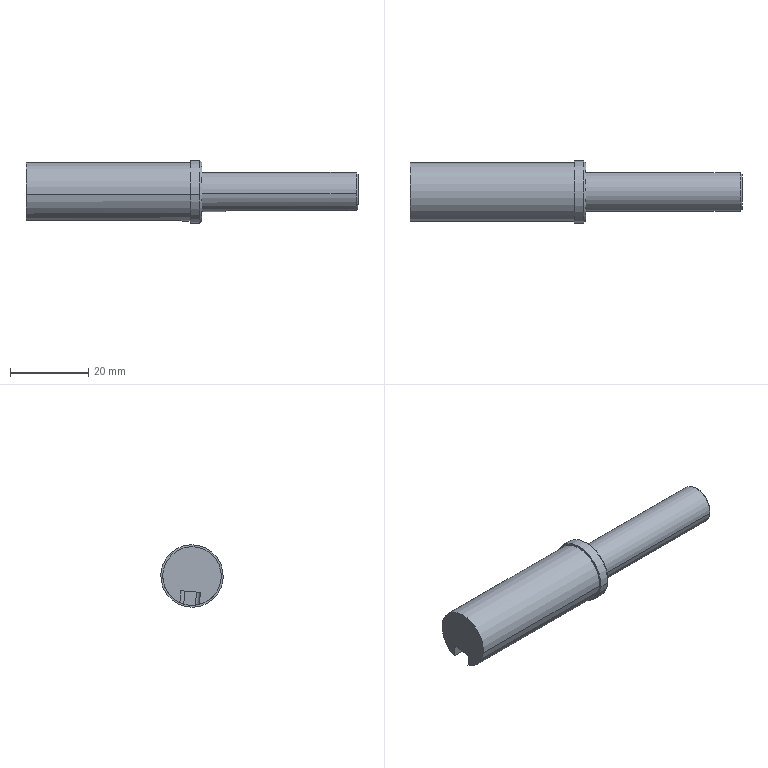Component | SolidWorks | 2018SOLIDWORKS1000000020-1 | 1 solid | 31 faces | box 85 x 16 x 16 mm | volume 10078 mm3 | cylinder 12 | plane 12 | cone 7 | commonest cylinder face diameters 2 x4 15 x2 3.3 x2 10 x2 16 x2 | material 45 Steel
build123d program:
from build123d import *

# Parameters (mm, degrees)
SKETCH1_R             = 8
BOSS_EXTRUDE1_DEPTH   = 45
SKETCH3_R             = 5
BOSS_EXTRUDE3_DEPTH   = 40
CHAMFER1_SIZE         = 0.5
M4_TAPPED_HOLE1_D     = 3.3
M4_TAPPED_HOLE1_DEPTH = 10
M4_TAPPED_HOLE1_TIP   = 0.9914
CHAMFER2_SIZE         = 0.5
SKETCH9_R             = 10
SKETCH9_R_2           = 7.5
CUT_EXTRUDE1_DEPTH    = 42
SKETCH10_W            = 5
SKETCH10_H            = 5
CUT_EXTRUDE2_DEPTH    = 40
FILLET1_R             = 1
SKETCH11_W            = 4
SKETCH11_H            = 4
CUT_EXTRUDE3_DEPTH    = 34
FILLET2_R             = 1


with BuildPart() as part:
    # Sketch1 → Boss-Extrude1 (new body)
    with BuildSketch(Plane.XY):
        with Locations(Location((0, 0, 0), (0, 0, 180))):
            Circle(SKETCH1_R)
    extrude(amount=BOSS_EXTRUDE1_DEPTH)

    # Sketch3 → Boss-Extrude3 (add)
    with BuildSketch(Plane.XY.offset(45)):
        Circle(SKETCH3_R)
    extrude(amount=BOSS_EXTRUDE3_DEPTH)

    # Chamfer1
    chamfer1_edges = [part.edges().sort_by_distance(p)[0] for p in [
        (8, 0, 0),
        (8, 0, 45),
    ]]
    chamfer(chamfer1_edges, length=CHAMFER1_SIZE)

    # M4 Tapped Hole1
    with Locations(Plane(origin=(0, 0, 85), x_dir=(-1, 0, 0), z_dir=(0, 0, 1))):
        with Locations((0, 0)):
            Hole(M4_TAPPED_HOLE1_D / 2, depth=M4_TAPPED_HOLE1_DEPTH)
            with Locations((0, 0, -(M4_TAPPED_HOLE1_DEPTH + M4_TAPPED_HOLE1_TIP / 2))):  # 118° drill point
                Cone(0, M4_TAPPED_HOLE1_D / 2, M4_TAPPED_HOLE1_TIP, mode=Mode.SUBTRACT)

    # Chamfer2
    chamfer2_edges = [part.edges().sort_by_distance(p)[0] for p in [
        (-5, 0, 85),
    ]]
    chamfer(chamfer2_edges, length=CHAMFER2_SIZE)

    # Sketch9 → Cut-Extrude1 (cut)
    with BuildSketch(Plane(origin=(0, 0, 0), x_dir=(-1, 0, 0), z_dir=(0, 0, -1))):
        Circle(SKETCH9_R)
        Circle(SKETCH9_R_2, mode=Mode.SUBTRACT)
    extrude(amount=-CUT_EXTRUDE1_DEPTH, mode=Mode.SUBTRACT)

    # Sketch10 → Cut-Extrude2 (cut)
    with BuildSketch(Plane(origin=(0, 0, 0), x_dir=(-1, 0, 0), z_dir=(0, 0, -1))):
        with Locations((0, 6.5)):
            Rectangle(SKETCH10_W, SKETCH10_H)
    extrude(amount=-CUT_EXTRUDE2_DEPTH, mode=Mode.SUBTRACT)

    # Fillet1
    fillet1_edges = [part.edges().sort_by_distance(p)[0] for p in [
        (2.5, 5.536, 40),
        (-2.5, 5.536, 40),
    ]]
    fillet(fillet1_edges, radius=FILLET1_R)

    # Sketch11 → Cut-Extrude3 (cut)
    with BuildSketch(Plane.XY.offset(85)):
        with Locations((0, 4.5)):
            Rectangle(SKETCH11_W, SKETCH11_H)
    extrude(amount=-CUT_EXTRUDE3_DEPTH, mode=Mode.SUBTRACT)

    # Fillet2
    fillet2_edges = [part.edges().sort_by_distance(p)[0] for p in [
        (-2, 3.541, 51),
        (2, 3.541, 51),
    ]]
    fillet(fillet2_edges, radius=FILLET2_R)


solid = part.part

# Placed as in the assembly
solid = solid.moved(Location((-72.284, -95.825, 207.018), (-85.06, 90, 0)))
STEP:
#1=COLOUR_RGB('',0.7922,0.8196,0.9333);
#2=FILL_AREA_STYLE_COLOUR('',#1);
#3=FILL_AREA_STYLE('',(#2));
#4=SURFACE_STYLE_FILL_AREA(#3);
#5=SURFACE_SIDE_STYLE('',(#4));
#6=SURFACE_STYLE_USAGE(.BOTH.,#5);
#7=PRESENTATION_STYLE_ASSIGNMENT((#6));
#8=CARTESIAN_POINT('',(-1.192,-3.478,8.176));
#9=VERTEX_POINT('',#8);
#10=CARTESIAN_POINT('',(-1.192,-4.067,8.125));
#11=VERTEX_POINT('',#10);
#12=CARTESIAN_POINT('',(-1.192,-3.773,8.15));
#13=DIRECTION('',(-1.,-0.,0.));
#14=DIRECTION('',(0.,-0.9963,-0.08611));
#15=AXIS2_PLACEMENT_3D('',#12,#13,#14);
#16=CIRCLE('',#15,0.2953);
#17=EDGE_CURVE('',#9,#11,#16,.T.);
#18=ORIENTED_EDGE('',*,*,#17,.T.);
#19=CARTESIAN_POINT('',(-2.846,-4.067,8.125));
#20=VERTEX_POINT('',#19);
#21=CARTESIAN_POINT('',(0.03939,-4.067,8.125));
#22=DIRECTION('',(-1.,-0.,0.));
#23=VECTOR('',#22,39.37);
#24=LINE('',#21,#23);
#25=EDGE_CURVE('',#11,#20,#24,.T.);
#26=ORIENTED_EDGE('',*,*,#25,.T.);
#27=CARTESIAN_POINT('',(-2.846,-3.847,7.864));
#28=VERTEX_POINT('',#27);
#29=CARTESIAN_POINT('',(-2.846,-3.773,8.15));
#30=DIRECTION('',(-1.,-0.,0.));
#31=DIRECTION('',(0.,0.9963,0.08611));
#32=AXIS2_PLACEMENT_3D('',#29,#30,#31);
#33=CIRCLE('',#32,0.2953);
#34=EDGE_CURVE('',#28,#20,#33,.T.);
#35=ORIENTED_EDGE('',*,*,#34,.F.);
#36=CARTESIAN_POINT('',(-1.31,-3.847,7.864));
#37=VERTEX_POINT('',#36);
#38=CARTESIAN_POINT('',(0.03939,-3.847,7.864));
#39=DIRECTION('',(-1.,-0.,0.));
#40=VECTOR('',#39,39.37);
#41=LINE('',#38,#40);
#42=EDGE_CURVE('',#37,#28,#41,.T.);
#43=ORIENTED_EDGE('',*,*,#42,.F.);
#44=CARTESIAN_POINT('',(-1.271,-3.807,7.857));
#45=VERTEX_POINT('',#44);
#46=CARTESIAN_POINT('',(-1.31,-3.847,7.864));
#47=CARTESIAN_POINT('',(-1.305,-3.847,7.864));
#48=CARTESIAN_POINT('',(-1.3,-3.846,7.864));
#49=CARTESIAN_POINT('',(-1.29,-3.841,7.863));
#50=CARTESIAN_POINT('',(-1.286,-3.838,7.862));
#51=CARTESIAN_POINT('',(-1.279,-3.831,7.861));
#52=CARTESIAN_POINT('',(-1.276,-3.827,7.86));
#53=CARTESIAN_POINT('',(-1.272,-3.817,7.858));
#54=CARTESIAN_POINT('',(-1.271,-3.812,7.858));
#55=CARTESIAN_POINT('',(-1.271,-3.807,7.857));
#56=B_SPLINE_CURVE_WITH_KNOTS('',3,(#46,#47,#48,#49,#50,#51,#52,#53,#54,#55),.UNSPECIFIED.,.F.,.F.,(4,2,2,2,4),(0.,0.0003975,0.000795,0.001193,0.00159),.UNSPECIFIED.);
#57=EDGE_CURVE('',#37,#45,#56,.T.);
#58=ORIENTED_EDGE('',*,*,#57,.T.);
#59=CARTESIAN_POINT('',(-1.271,-3.689,7.867));
#60=VERTEX_POINT('',#59);
#61=CARTESIAN_POINT('',(-1.271,-3.773,8.15));
#62=DIRECTION('',(1.,0.,-0.));
#63=DIRECTION('',(0.,0.9963,0.08611));
#64=AXIS2_PLACEMENT_3D('',#61,#62,#63);
#65=CIRCLE('',#64,0.2953);
#66=EDGE_CURVE('',#45,#60,#65,.T.);
#67=ORIENTED_EDGE('',*,*,#66,.T.);
#68=CARTESIAN_POINT('',(-1.31,-3.651,7.881));
#69=VERTEX_POINT('',#68);
#70=CARTESIAN_POINT('',(-1.271,-3.689,7.867));
#71=CARTESIAN_POINT('',(-1.271,-3.684,7.869));
#72=CARTESIAN_POINT('',(-1.272,-3.679,7.87));
#73=CARTESIAN_POINT('',(-1.276,-3.67,7.874));
#74=CARTESIAN_POINT('',(-1.279,-3.665,7.875));
#75=CARTESIAN_POINT('',(-1.286,-3.658,7.878));
#76=CARTESIAN_POINT('',(-1.29,-3.656,7.879));
#77=CARTESIAN_POINT('',(-1.3,-3.652,7.881));
#78=CARTESIAN_POINT('',(-1.305,-3.651,7.881));
#79=CARTESIAN_POINT('',(-1.31,-3.651,7.881));
#80=B_SPLINE_CURVE_WITH_KNOTS('',3,(#70,#71,#72,#73,#74,#75,#76,#77,#78,#79),.UNSPECIFIED.,.F.,.F.,(4,2,2,2,4),(0.,0.0003975,0.000795,0.001193,0.00159),.UNSPECIFIED.);
#81=EDGE_CURVE('',#60,#69,#80,.T.);
#82=ORIENTED_EDGE('',*,*,#81,.T.);
#83=CARTESIAN_POINT('',(-2.846,-3.651,7.881));
#84=VERTEX_POINT('',#83);
#85=CARTESIAN_POINT('',(0.03939,-3.651,7.881));
#86=DIRECTION('',(1.,0.,-0.));
#87=VECTOR('',#86,39.37);
#88=LINE('',#85,#87);
#89=EDGE_CURVE('',#84,#69,#88,.T.);
#90=ORIENTED_EDGE('',*,*,#89,.F.);
#91=CARTESIAN_POINT('',(-2.846,-3.478,8.176));
#92=VERTEX_POINT('',#91);
#93=CARTESIAN_POINT('',(-2.846,-3.773,8.15));
#94=DIRECTION('',(-1.,-0.,0.));
#95=DIRECTION('',(0.,0.9963,0.08611));
#96=AXIS2_PLACEMENT_3D('',#93,#94,#95);
#97=CIRCLE('',#96,0.2953);
#98=EDGE_CURVE('',#92,#84,#97,.T.);
#99=ORIENTED_EDGE('',*,*,#98,.F.);
#100=CARTESIAN_POINT('',(0.03939,-3.478,8.176));
#101=DIRECTION('',(-1.,-0.,0.));
#102=VECTOR('',#101,39.37);
#103=LINE('',#100,#102);
#104=EDGE_CURVE('',#9,#92,#103,.T.);
#105=ORIENTED_EDGE('',*,*,#104,.F.);
#106=EDGE_LOOP('',(#18,#26,#35,#43,#58,#67,#82,#90,#99,#105));
#107=FACE_OUTER_BOUND('',#106,.T.);
#108=CARTESIAN_POINT('',(0.03939,-3.773,8.15));
#109=DIRECTION('',(-1.,-0.,0.));
#110=DIRECTION('',(-0.,0.9963,0.08611));
#111=AXIS2_PLACEMENT_3D('',#108,#109,#110);
#112=CYLINDRICAL_SURFACE('',#111,0.2953);
#113=ADVANCED_FACE('',(#107),#112,.T.);
#114=CARTESIAN_POINT('',(0.5006,-3.949,8.135));
#115=VERTEX_POINT('',#114);
#116=CARTESIAN_POINT('',(0.5006,-3.837,7.985));
#117=VERTEX_POINT('',#116);
#118=CARTESIAN_POINT('',(0.5006,-3.773,8.15));
#119=DIRECTION('',(1.,0.,-0.));
#120=DIRECTION('',(0.,-0.9963,-0.08611));
#121=AXIS2_PLACEMENT_3D('',#118,#119,#120);
#122=CIRCLE('',#121,0.1772);
#123=EDGE_CURVE('',#115,#117,#122,.T.);
#124=ORIENTED_EDGE('',*,*,#123,.F.);
#125=CARTESIAN_POINT('',(0.481,-3.969,8.133));
#126=VERTEX_POINT('',#125);
#127=CARTESIAN_POINT('',(0.5006,-3.949,8.135));
#128=DIRECTION('',(-0.7071,-0.7045,-0.06089));
#129=VECTOR('',#128,39.37);
#130=LINE('',#127,#129);
#131=EDGE_CURVE('',#115,#126,#130,.T.);
#132=ORIENTED_EDGE('',*,*,#131,.T.);
#133=CARTESIAN_POINT('',(0.481,-3.836,7.964));
#134=VERTEX_POINT('',#133);
#135=CARTESIAN_POINT('',(0.481,-3.773,8.15));
#136=DIRECTION('',(-1.,-0.,0.));
#137=DIRECTION('',(0.,-0.9963,-0.08611));
#138=AXIS2_PLACEMENT_3D('',#135,#136,#137);
#139=CIRCLE('',#138,0.1969);
#140=EDGE_CURVE('',#134,#126,#139,.T.);
#141=ORIENTED_EDGE('',*,*,#140,.F.);
#142=CARTESIAN_POINT('',(0.5006,-3.837,7.985));
#143=CARTESIAN_POINT('',(0.4941,-3.837,7.978));
#144=CARTESIAN_POINT('',(0.4876,-3.836,7.971));
#145=CARTESIAN_POINT('',(0.481,-3.836,7.964));
#146=B_SPLINE_CURVE_WITH_KNOTS('',3,(#142,#143,#144,#145),.UNSPECIFIED.,.F.,.F.,(4,4),(0.002374,0.003118),.UNSPECIFIED.);
#147=EDGE_CURVE('',#117,#134,#146,.T.);
#148=ORIENTED_EDGE('',*,*,#147,.F.);
#149=EDGE_LOOP('',(#124,#132,#141,#148));
#150=FACE_OUTER_BOUND('',#149,.T.);
#151=CARTESIAN_POINT('',(0.5006,-3.773,8.15));
#152=DIRECTION('',(-1.,-0.,0.));
#153=DIRECTION('',(-0.,0.9963,0.08611));
#154=AXIS2_PLACEMENT_3D('',#151,#152,#153);
#155=CONICAL_SURFACE('',#154,0.1772,0.7854);
#156=ADVANCED_FACE('',(#150),#155,.T.);
#157=ORIENTED_EDGE('',*,*,#131,.F.);
#158=CARTESIAN_POINT('',(0.5006,-3.596,8.166));
#159=VERTEX_POINT('',#158);
#160=CARTESIAN_POINT('',(0.5006,-3.773,8.15));
#161=DIRECTION('',(1.,0.,-0.));
#162=DIRECTION('',(0.,-0.9963,-0.08611));
#163=AXIS2_PLACEMENT_3D('',#160,#161,#162);
#164=CIRCLE('',#163,0.1772);
#165=EDGE_CURVE('',#159,#115,#164,.T.);
#166=ORIENTED_EDGE('',*,*,#165,.F.);
#167=CARTESIAN_POINT('',(0.481,-3.577,8.167));
#168=VERTEX_POINT('',#167);
#169=CARTESIAN_POINT('',(0.5006,-3.596,8.166));
#170=DIRECTION('',(-0.7071,0.7045,0.06089));
#171=VECTOR('',#170,39.37);
#172=LINE('',#169,#171);
#173=EDGE_CURVE('',#159,#168,#172,.T.);
#174=ORIENTED_EDGE('',*,*,#173,.T.);
#175=CARTESIAN_POINT('',(0.481,-3.773,8.15));
#176=DIRECTION('',(-1.,-0.,0.));
#177=DIRECTION('',(0.,-0.9963,-0.08611));
#178=AXIS2_PLACEMENT_3D('',#175,#176,#177);
#179=CIRCLE('',#178,0.1969);
#180=EDGE_CURVE('',#126,#168,#179,.T.);
#181=ORIENTED_EDGE('',*,*,#180,.F.);
#182=EDGE_LOOP('',(#157,#166,#174,#181));
#183=FACE_OUTER_BOUND('',#182,.T.);
#184=CARTESIAN_POINT('',(0.5006,-3.773,8.15));
#185=DIRECTION('',(-1.,-0.,0.));
#186=DIRECTION('',(-0.,0.9963,0.08611));
#187=AXIS2_PLACEMENT_3D('',#184,#185,#186);
#188=CONICAL_SURFACE('',#187,0.1772,0.7854);
#189=ADVANCED_FACE('',(#183),#188,.T.);
#190=CARTESIAN_POINT('',(0.1069,-3.708,8.156));
#191=VERTEX_POINT('',#190);
#192=CARTESIAN_POINT('',(0.1069,-3.837,8.145));
#193=VERTEX_POINT('',#192);
#194=CARTESIAN_POINT('',(0.1069,-3.773,8.15));
#195=DIRECTION('',(1.,0.,-0.));
#196=DIRECTION('',(0.,-0.9963,-0.08611));
#197=AXIS2_PLACEMENT_3D('',#194,#195,#196);
#198=CIRCLE('',#197,0.06496);
#199=EDGE_CURVE('',#191,#193,#198,.T.);
#200=ORIENTED_EDGE('',*,*,#199,.F.);
#201=CARTESIAN_POINT('',(0.5006,-3.708,8.156));
#202=VERTEX_POINT('',#201);
#203=CARTESIAN_POINT('',(0.5006,-3.708,8.156));
#204=DIRECTION('',(1.,0.,-0.));
#205=VECTOR('',#204,39.37);
#206=LINE('',#203,#205);
#207=EDGE_CURVE('',#191,#202,#206,.T.);
#208=ORIENTED_EDGE('',*,*,#207,.T.);
#209=CARTESIAN_POINT('',(0.5006,-3.837,8.145));
#210=VERTEX_POINT('',#209);
#211=CARTESIAN_POINT('',(0.5006,-3.773,8.15));
#212=DIRECTION('',(1.,0.,-0.));
#213=DIRECTION('',(0.,-0.9963,-0.08611));
#214=AXIS2_PLACEMENT_3D('',#211,#212,#213);
#215=CIRCLE('',#214,0.06496);
#216=EDGE_CURVE('',#202,#210,#215,.T.);
#217=ORIENTED_EDGE('',*,*,#216,.T.);
#218=CARTESIAN_POINT('',(0.5006,-3.837,8.145));
#219=DIRECTION('',(1.,0.,-0.));
#220=VECTOR('',#219,39.37);
#221=LINE('',#218,#220);
#222=EDGE_CURVE('',#193,#210,#221,.T.);
#223=ORIENTED_EDGE('',*,*,#222,.F.);
#224=EDGE_LOOP('',(#200,#208,#217,#223));
#225=FACE_OUTER_BOUND('',#224,.T.);
#226=CARTESIAN_POINT('',(0.5006,-3.773,8.15));
#227=DIRECTION('',(1.,0.,-0.));
#228=DIRECTION('',(0.,-0.9963,-0.08611));
#229=AXIS2_PLACEMENT_3D('',#226,#227,#228);
#230=CYLINDRICAL_SURFACE('',#229,0.06496);
#231=ADVANCED_FACE('',(#225),#230,.F.);
#232=CARTESIAN_POINT('',(0.06791,-3.773,8.15));
#233=VERTEX_POINT('',#232);
#234=CARTESIAN_POINT('',(0.1069,-3.837,8.145));
#235=DIRECTION('',(0.515,-0.854,-0.07381));
#236=VECTOR('',#235,39.37);
#237=LINE('',#234,#236);
#238=EDGE_CURVE('',#233,#193,#237,.T.);
#239=ORIENTED_EDGE('',*,*,#238,.F.);
#240=CARTESIAN_POINT('',(0.1069,-3.708,8.156));
#241=DIRECTION('',(0.515,0.854,0.07381));
#242=VECTOR('',#241,39.37);
#243=LINE('',#240,#242);
#244=EDGE_CURVE('',#233,#191,#243,.T.);
#245=ORIENTED_EDGE('',*,*,#244,.T.);
#246=ORIENTED_EDGE('',*,*,#199,.T.);
#247=EDGE_LOOP('',(#239,#245,#246));
#248=FACE_OUTER_BOUND('',#247,.T.);
#249=CARTESIAN_POINT('',(0.1069,-3.773,8.15));
#250=DIRECTION('',(1.,0.,-0.));
#251=DIRECTION('',(0.,-0.9963,-0.08611));
#252=AXIS2_PLACEMENT_3D('',#249,#250,#251);
#253=CONICAL_SURFACE('',#252,0.06496,1.03);
#254=ADVANCED_FACE('',(#248),#253,.F.);
#255=CARTESIAN_POINT('',(-1.074,-4.067,8.125));
#256=VERTEX_POINT('',#255);
#257=CARTESIAN_POINT('',(-1.074,-3.478,8.176));
#258=VERTEX_POINT('',#257);
#259=CARTESIAN_POINT('',(-1.074,-3.773,8.15));
#260=DIRECTION('',(1.,0.,-0.));
#261=DIRECTION('',(0.,-0.9963,-0.08611));
#262=AXIS2_PLACEMENT_3D('',#259,#260,#261);
#263=CIRCLE('',#262,0.2953);
#264=EDGE_CURVE('',#256,#258,#263,.T.);
#265=ORIENTED_EDGE('',*,*,#264,.F.);
#266=CARTESIAN_POINT('',(-1.094,-4.086,8.123));
#267=VERTEX_POINT('',#266);
#268=CARTESIAN_POINT('',(-1.074,-4.067,8.125));
#269=DIRECTION('',(-0.7071,-0.7045,-0.06089));
#270=VECTOR('',#269,39.37);
#271=LINE('',#268,#270);
#272=EDGE_CURVE('',#256,#267,#271,.T.);
#273=ORIENTED_EDGE('',*,*,#272,.T.);
#274=CARTESIAN_POINT('',(-1.094,-3.459,8.177));
#275=VERTEX_POINT('',#274);
#276=CARTESIAN_POINT('',(-1.094,-3.773,8.15));
#277=DIRECTION('',(-1.,-0.,0.));
#278=DIRECTION('',(0.,-0.9963,-0.08611));
#279=AXIS2_PLACEMENT_3D('',#276,#277,#278);
#280=CIRCLE('',#279,0.315);
#281=EDGE_CURVE('',#275,#267,#280,.T.);
#282=ORIENTED_EDGE('',*,*,#281,.F.);
#283=CARTESIAN_POINT('',(-1.074,-3.478,8.176));
#284=DIRECTION('',(-0.7071,0.7045,0.06089));
#285=VECTOR('',#284,39.37);
#286=LINE('',#283,#285);
#287=EDGE_CURVE('',#258,#275,#286,.T.);
#288=ORIENTED_EDGE('',*,*,#287,.F.);
#289=EDGE_LOOP('',(#265,#273,#282,#288));
#290=FACE_OUTER_BOUND('',#289,.T.);
#291=CARTESIAN_POINT('',(-1.074,-3.773,8.15));
#292=DIRECTION('',(-1.,-0.,0.));
#293=DIRECTION('',(-0.,0.9963,0.08611));
#294=AXIS2_PLACEMENT_3D('',#291,#292,#293);
#295=CONICAL_SURFACE('',#294,0.2953,0.7854);
#296=ADVANCED_FACE('',(#290),#295,.T.);
#297=ORIENTED_EDGE('',*,*,#140,.T.);
#298=CARTESIAN_POINT('',(-1.074,-3.969,8.133));
#299=VERTEX_POINT('',#298);
#300=CARTESIAN_POINT('',(0.5006,-3.969,8.133));
#301=DIRECTION('',(-1.,-0.,0.));
#302=VECTOR('',#301,39.37);
#303=LINE('',#300,#302);
#304=EDGE_CURVE('',#126,#299,#303,.T.);
#305=ORIENTED_EDGE('',*,*,#304,.T.);
#306=CARTESIAN_POINT('',(-1.074,-3.577,8.167));
#307=VERTEX_POINT('',#306);
#308=CARTESIAN_POINT('',(-1.074,-3.773,8.15));
#309=DIRECTION('',(1.,0.,-0.));
#310=DIRECTION('',(0.,-0.9963,-0.08611));
#311=AXIS2_PLACEMENT_3D('',#308,#309,#310);
#312=CIRCLE('',#311,0.1969);
#313=EDGE_CURVE('',#299,#307,#312,.T.);
#314=ORIENTED_EDGE('',*,*,#313,.T.);
#315=CARTESIAN_POINT('',(0.5006,-3.577,8.167));
#316=DIRECTION('',(-1.,-0.,0.));
#317=VECTOR('',#316,39.37);
#318=LINE('',#315,#317);
#319=EDGE_CURVE('',#168,#307,#318,.T.);
#320=ORIENTED_EDGE('',*,*,#319,.F.);
#321=CARTESIAN_POINT('',(0.481,-3.679,7.977));
#322=VERTEX_POINT('',#321);
#323=CARTESIAN_POINT('',(0.481,-3.773,8.15));
#324=DIRECTION('',(-1.,-0.,0.));
#325=DIRECTION('',(0.,-0.9963,-0.08611));
#326=AXIS2_PLACEMENT_3D('',#323,#324,#325);
#327=CIRCLE('',#326,0.1969);
#328=EDGE_CURVE('',#168,#322,#327,.T.);
#329=ORIENTED_EDGE('',*,*,#328,.T.);
#330=CARTESIAN_POINT('',(-0.7986,-3.679,7.977));
#331=VERTEX_POINT('',#330);
#332=CARTESIAN_POINT('',(0.5006,-3.679,7.977));
#333=DIRECTION('',(-1.,-0.,0.));
#334=VECTOR('',#333,39.37);
#335=LINE('',#332,#334);
#336=EDGE_CURVE('',#322,#331,#335,.T.);
#337=ORIENTED_EDGE('',*,*,#336,.T.);
#338=CARTESIAN_POINT('',(-0.8379,-3.717,7.962));
#339=VERTEX_POINT('',#338);
#340=CARTESIAN_POINT('',(-0.7986,-3.679,7.977));
#341=CARTESIAN_POINT('',(-0.8039,-3.679,7.977));
#342=CARTESIAN_POINT('',(-0.8091,-3.68,7.977));
#343=CARTESIAN_POINT('',(-0.8187,-3.684,7.975));
#344=CARTESIAN_POINT('',(-0.823,-3.686,7.973));
#345=CARTESIAN_POINT('',(-0.8302,-3.693,7.97));
#346=CARTESIAN_POINT('',(-0.833,-3.698,7.968));
#347=CARTESIAN_POINT('',(-0.8369,-3.707,7.965));
#348=CARTESIAN_POINT('',(-0.8379,-3.712,7.963));
#349=CARTESIAN_POINT('',(-0.8379,-3.717,7.962));
#350=B_SPLINE_CURVE_WITH_KNOTS('',3,(#340,#341,#342,#343,#344,#345,#346,#347,#348,#349),.UNSPECIFIED.,.F.,.F.,(4,2,2,2,4),(0.,0.0003995,0.0007989,0.001198,0.001598),.UNSPECIFIED.);
#351=EDGE_CURVE('',#331,#339,#350,.T.);
#352=ORIENTED_EDGE('',*,*,#351,.T.);
#353=CARTESIAN_POINT('',(-0.8379,-3.795,7.955));
#354=VERTEX_POINT('',#353);
#355=CARTESIAN_POINT('',(-0.8379,-3.773,8.15));
#356=DIRECTION('',(1.,0.,-0.));
#357=DIRECTION('',(0.,-0.9963,-0.08611));
#358=AXIS2_PLACEMENT_3D('',#355,#356,#357);
#359=CIRCLE('',#358,0.1969);
#360=EDGE_CURVE('',#354,#339,#359,.T.);
#361=ORIENTED_EDGE('',*,*,#360,.F.);
#362=CARTESIAN_POINT('',(-0.7986,-3.836,7.964));
#363=VERTEX_POINT('',#362);
#364=CARTESIAN_POINT('',(-0.8379,-3.795,7.955));
#365=CARTESIAN_POINT('',(-0.8379,-3.801,7.955));
#366=CARTESIAN_POINT('',(-0.8369,-3.806,7.956));
#367=CARTESIAN_POINT('',(-0.833,-3.815,7.958));
#368=CARTESIAN_POINT('',(-0.8302,-3.82,7.959));
#369=CARTESIAN_POINT('',(-0.823,-3.827,7.961));
#370=CARTESIAN_POINT('',(-0.8187,-3.83,7.962));
#371=CARTESIAN_POINT('',(-0.8092,-3.834,7.963));
#372=CARTESIAN_POINT('',(-0.8039,-3.836,7.964));
#373=CARTESIAN_POINT('',(-0.7986,-3.836,7.964));
#374=B_SPLINE_CURVE_WITH_KNOTS('',3,(#364,#365,#366,#367,#368,#369,#370,#371,#372,#373),.UNSPECIFIED.,.F.,.F.,(4,2,2,2,4),(0.,0.0003995,0.0007989,0.001198,0.001598),.UNSPECIFIED.);
#375=EDGE_CURVE('',#354,#363,#374,.T.);
#376=ORIENTED_EDGE('',*,*,#375,.T.);
#377=CARTESIAN_POINT('',(0.5006,-3.836,7.964));
#378=DIRECTION('',(1.,0.,-0.));
#379=VECTOR('',#378,39.37);
#380=LINE('',#377,#379);
#381=EDGE_CURVE('',#363,#134,#380,.T.);
#382=ORIENTED_EDGE('',*,*,#381,.T.);
#383=EDGE_LOOP('',(#297,#305,#314,#320,#329,#337,#352,#361,#376,#382));
#384=FACE_OUTER_BOUND('',#383,.T.);
#385=CARTESIAN_POINT('',(0.5006,-3.773,8.15));
#386=DIRECTION('',(-1.,-0.,0.));
#387=DIRECTION('',(-0.,0.9963,0.08611));
#388=AXIS2_PLACEMENT_3D('',#385,#386,#387);
#389=CYLINDRICAL_SURFACE('',#388,0.1969);
#390=ADVANCED_FACE('',(#384),#389,.T.);
#391=ORIENTED_EDGE('',*,*,#281,.T.);
#392=CARTESIAN_POINT('',(-1.192,-4.086,8.123));
#393=VERTEX_POINT('',#392);
#394=CARTESIAN_POINT('',(-1.074,-4.086,8.123));
#395=DIRECTION('',(-1.,-0.,0.));
#396=VECTOR('',#395,39.37);
#397=LINE('',#394,#396);
#398=EDGE_CURVE('',#267,#393,#397,.T.);
#399=ORIENTED_EDGE('',*,*,#398,.T.);
#400=CARTESIAN_POINT('',(-1.192,-3.459,8.177));
#401=VERTEX_POINT('',#400);
#402=CARTESIAN_POINT('',(-1.192,-3.773,8.15));
#403=DIRECTION('',(1.,0.,-0.));
#404=DIRECTION('',(0.,-0.9963,-0.08611));
#405=AXIS2_PLACEMENT_3D('',#402,#403,#404);
#406=CIRCLE('',#405,0.315);
#407=EDGE_CURVE('',#393,#401,#406,.T.);
#408=ORIENTED_EDGE('',*,*,#407,.T.);
#409=CARTESIAN_POINT('',(-1.074,-3.459,8.177));
#410=DIRECTION('',(-1.,-0.,0.));
#411=VECTOR('',#410,39.37);
#412=LINE('',#409,#411);
#413=EDGE_CURVE('',#275,#401,#412,.T.);
#414=ORIENTED_EDGE('',*,*,#413,.F.);
#415=EDGE_LOOP('',(#391,#399,#408,#414));
#416=FACE_OUTER_BOUND('',#415,.T.);
#417=CARTESIAN_POINT('',(-1.074,-3.773,8.15));
#418=DIRECTION('',(-1.,-0.,0.));
#419=DIRECTION('',(-0.,0.9963,0.08611));
#420=AXIS2_PLACEMENT_3D('',#417,#418,#419);
#421=CYLINDRICAL_SURFACE('',#420,0.315);
#422=ADVANCED_FACE('',(#416),#421,.T.);
#423=CARTESIAN_POINT('',(-1.074,-3.773,8.15));
#424=DIRECTION('',(1.,0.,-0.));
#425=DIRECTION('',(0.,-0.9963,-0.08611));
#426=AXIS2_PLACEMENT_3D('',#423,#424,#425);
#427=CIRCLE('',#426,0.2953);
#428=EDGE_CURVE('',#258,#256,#427,.T.);
#429=ORIENTED_EDGE('',*,*,#428,.T.);
#430=ORIENTED_EDGE('',*,*,#264,.T.);
#431=EDGE_LOOP('',(#429,#430));
#432=FACE_OUTER_BOUND('',#431,.T.);
#433=CARTESIAN_POINT('',(-1.074,-3.773,8.15));
#434=DIRECTION('',(1.,0.,-0.));
#435=DIRECTION('',(0.,-0.9963,-0.08611));
#436=AXIS2_PLACEMENT_3D('',#433,#434,#435);
#437=CIRCLE('',#436,0.1969);
#438=EDGE_CURVE('',#307,#299,#437,.T.);
#439=ORIENTED_EDGE('',*,*,#438,.F.);
#440=ORIENTED_EDGE('',*,*,#313,.F.);
#441=EDGE_LOOP('',(#439,#440));
#442=FACE_BOUND('',#441,.T.);
#443=CARTESIAN_POINT('',(-1.074,-3.773,8.15));
#444=DIRECTION('',(1.,0.,-0.));
#445=DIRECTION('',(0.,-0.9963,-0.08611));
#446=AXIS2_PLACEMENT_3D('',#443,#444,#445);
#447=PLANE('',#446);
#448=ADVANCED_FACE('',(#432,#442),#447,.T.);
#449=ORIENTED_EDGE('',*,*,#398,.F.);
#450=CARTESIAN_POINT('',(-1.094,-3.773,8.15));
#451=DIRECTION('',(-1.,-0.,0.));
#452=DIRECTION('',(0.,-0.9963,-0.08611));
#453=AXIS2_PLACEMENT_3D('',#450,#451,#452);
#454=CIRCLE('',#453,0.315);
#455=EDGE_CURVE('',#267,#275,#454,.T.);
#456=ORIENTED_EDGE('',*,*,#455,.T.);
#457=ORIENTED_EDGE('',*,*,#413,.T.);
#458=CARTESIAN_POINT('',(-1.192,-3.773,8.15));
#459=DIRECTION('',(1.,0.,-0.));
#460=DIRECTION('',(0.,-0.9963,-0.08611));
#461=AXIS2_PLACEMENT_3D('',#458,#459,#460);
#462=CIRCLE('',#461,0.315);
#463=EDGE_CURVE('',#401,#393,#462,.T.);
#464=ORIENTED_EDGE('',*,*,#463,.T.);
#465=EDGE_LOOP('',(#449,#456,#457,#464));
#466=FACE_OUTER_BOUND('',#465,.T.);
#467=CARTESIAN_POINT('',(-1.074,-3.773,8.15));
#468=DIRECTION('',(-1.,-0.,0.));
#469=DIRECTION('',(-0.,0.9963,0.08611));
#470=AXIS2_PLACEMENT_3D('',#467,#468,#469);
#471=CYLINDRICAL_SURFACE('',#470,0.315);
#472=ADVANCED_FACE('',(#466),#471,.T.);
#473=ORIENTED_EDGE('',*,*,#304,.F.);
#474=ORIENTED_EDGE('',*,*,#180,.T.);
#475=ORIENTED_EDGE('',*,*,#319,.T.);
#476=ORIENTED_EDGE('',*,*,#438,.T.);
#477=EDGE_LOOP('',(#473,#474,#475,#476));
#478=FACE_OUTER_BOUND('',#477,.T.);
#479=CARTESIAN_POINT('',(0.5006,-3.773,8.15));
#480=DIRECTION('',(-1.,-0.,0.));
#481=DIRECTION('',(-0.,0.9963,0.08611));
#482=AXIS2_PLACEMENT_3D('',#479,#480,#481);
#483=CYLINDRICAL_SURFACE('',#482,0.1969);
#484=ADVANCED_FACE('',(#478),#483,.T.);
#485=CARTESIAN_POINT('',(0.5006,-3.681,7.999));
#486=VERTEX_POINT('',#485);
#487=CARTESIAN_POINT('',(0.5006,-3.686,8.059));
#488=VERTEX_POINT('',#487);
#489=CARTESIAN_POINT('',(0.5006,-3.672,7.902));
#490=DIRECTION('',(0.,-0.08611,0.9963));
#491=VECTOR('',#490,39.37);
#492=LINE('',#489,#491);
#493=EDGE_CURVE('',#486,#488,#492,.T.);
#494=ORIENTED_EDGE('',*,*,#493,.F.);
#495=CARTESIAN_POINT('',(0.5006,-3.773,8.15));
#496=DIRECTION('',(1.,0.,-0.));
#497=DIRECTION('',(0.,-0.9963,-0.08611));
#498=AXIS2_PLACEMENT_3D('',#495,#496,#497);
#499=CIRCLE('',#498,0.1772);
#500=EDGE_CURVE('',#486,#159,#499,.T.);
#501=ORIENTED_EDGE('',*,*,#500,.T.);
#502=ORIENTED_EDGE('',*,*,#165,.T.);
#503=ORIENTED_EDGE('',*,*,#123,.T.);
#504=CARTESIAN_POINT('',(0.5006,-3.843,8.045));
#505=VERTEX_POINT('',#504);
#506=CARTESIAN_POINT('',(0.5006,-3.829,7.889));
#507=DIRECTION('',(-0.,0.08611,-0.9963));
#508=VECTOR('',#507,39.37);
#509=LINE('',#506,#508);
#510=EDGE_CURVE('',#505,#117,#509,.T.);
#511=ORIENTED_EDGE('',*,*,#510,.F.);
#512=CARTESIAN_POINT('',(0.5006,-3.686,8.059));
#513=DIRECTION('',(0.,-0.9963,-0.08611));
#514=VECTOR('',#513,39.37);
#515=LINE('',#512,#514);
#516=EDGE_CURVE('',#488,#505,#515,.T.);
#517=ORIENTED_EDGE('',*,*,#516,.F.);
#518=EDGE_LOOP('',(#494,#501,#502,#503,#511,#517));
#519=FACE_OUTER_BOUND('',#518,.T.);
#520=CARTESIAN_POINT('',(0.5006,-3.773,8.15));
#521=DIRECTION('',(1.,0.,-0.));
#522=DIRECTION('',(0.,-0.9963,-0.08611));
#523=AXIS2_PLACEMENT_3D('',#520,#521,#522);
#524=CIRCLE('',#523,0.06496);
#525=EDGE_CURVE('',#210,#202,#524,.T.);
#526=ORIENTED_EDGE('',*,*,#525,.F.);
#527=ORIENTED_EDGE('',*,*,#216,.F.);
#528=EDGE_LOOP('',(#526,#527));
#529=FACE_BOUND('',#528,.T.);
#530=CARTESIAN_POINT('',(0.5006,-3.773,8.15));
#531=DIRECTION('',(1.,0.,-0.));
#532=DIRECTION('',(0.,-0.9963,-0.08611));
#533=AXIS2_PLACEMENT_3D('',#530,#531,#532);
#534=PLANE('',#533);
#535=ADVANCED_FACE('',(#519,#529),#534,.T.);
#536=ORIENTED_EDGE('',*,*,#272,.F.);
#537=ORIENTED_EDGE('',*,*,#428,.F.);
#538=ORIENTED_EDGE('',*,*,#287,.T.);
#539=ORIENTED_EDGE('',*,*,#455,.F.);
#540=EDGE_LOOP('',(#536,#537,#538,#539));
#541=FACE_OUTER_BOUND('',#540,.T.);
#542=CARTESIAN_POINT('',(-1.074,-3.773,8.15));
#543=DIRECTION('',(-1.,-0.,0.));
#544=DIRECTION('',(-0.,0.9963,0.08611));
#545=AXIS2_PLACEMENT_3D('',#542,#543,#544);
#546=CONICAL_SURFACE('',#545,0.2953,0.7854);
#547=ADVANCED_FACE('',(#541),#546,.T.);
#548=ORIENTED_EDGE('',*,*,#244,.F.);
#549=ORIENTED_EDGE('',*,*,#238,.T.);
#550=CARTESIAN_POINT('',(0.1069,-3.773,8.15));
#551=DIRECTION('',(1.,0.,-0.));
#552=DIRECTION('',(0.,-0.9963,-0.08611));
#553=AXIS2_PLACEMENT_3D('',#550,#551,#552);
#554=CIRCLE('',#553,0.06496);
#555=EDGE_CURVE('',#193,#191,#554,.T.);
#556=ORIENTED_EDGE('',*,*,#555,.T.);
#557=EDGE_LOOP('',(#548,#549,#556));
#558=FACE_OUTER_BOUND('',#557,.T.);
#559=CARTESIAN_POINT('',(0.1069,-3.773,8.15));
#560=DIRECTION('',(1.,0.,-0.));
#561=DIRECTION('',(0.,-0.9963,-0.08611));
#562=AXIS2_PLACEMENT_3D('',#559,#560,#561);
#563=CONICAL_SURFACE('',#562,0.06496,1.03);
#564=ADVANCED_FACE('',(#558),#563,.F.);
#565=ORIENTED_EDGE('',*,*,#207,.F.);
#566=ORIENTED_EDGE('',*,*,#555,.F.);
#567=ORIENTED_EDGE('',*,*,#222,.T.);
#568=ORIENTED_EDGE('',*,*,#525,.T.);
#569=EDGE_LOOP('',(#565,#566,#567,#568));
#570=FACE_OUTER_BOUND('',#569,.T.);
#571=CARTESIAN_POINT('',(0.5006,-3.773,8.15));
#572=DIRECTION('',(1.,0.,-0.));
#573=DIRECTION('',(0.,-0.9963,-0.08611));
#574=AXIS2_PLACEMENT_3D('',#571,#572,#573);
#575=CYLINDRICAL_SURFACE('',#574,0.06496);
#576=ADVANCED_FACE('',(#570),#575,.F.);
#577=ORIENTED_EDGE('',*,*,#173,.F.);
#578=ORIENTED_EDGE('',*,*,#500,.F.);
#579=CARTESIAN_POINT('',(0.481,-3.679,7.977));
#580=CARTESIAN_POINT('',(0.4876,-3.679,7.985));
#581=CARTESIAN_POINT('',(0.4941,-3.68,7.992));
#582=CARTESIAN_POINT('',(0.5006,-3.681,7.999));
#583=B_SPLINE_CURVE_WITH_KNOTS('',3,(#579,#580,#581,#582),.UNSPECIFIED.,.F.,.F.,(4,4),(0.004191,0.004935),.UNSPECIFIED.);
#584=EDGE_CURVE('',#322,#486,#583,.T.);
#585=ORIENTED_EDGE('',*,*,#584,.F.);
#586=ORIENTED_EDGE('',*,*,#328,.F.);
#587=EDGE_LOOP('',(#577,#578,#585,#586));
#588=FACE_OUTER_BOUND('',#587,.T.);
#589=CARTESIAN_POINT('',(0.5006,-3.773,8.15));
#590=DIRECTION('',(-1.,-0.,0.));
#591=DIRECTION('',(-0.,0.9963,0.08611));
#592=AXIS2_PLACEMENT_3D('',#589,#590,#591);
#593=CONICAL_SURFACE('',#592,0.1772,0.7854);
#594=ADVANCED_FACE('',(#588),#593,.T.);
#595=ORIENTED_EDGE('',*,*,#17,.F.);
#596=CARTESIAN_POINT('',(-1.192,-3.773,8.15));
#597=DIRECTION('',(-1.,-0.,0.));
#598=DIRECTION('',(0.,-0.9963,-0.08611));
#599=AXIS2_PLACEMENT_3D('',#596,#597,#598);
#600=CIRCLE('',#599,0.2953);
#601=EDGE_CURVE('',#11,#9,#600,.T.);
#602=ORIENTED_EDGE('',*,*,#601,.F.);
#603=EDGE_LOOP('',(#595,#602));
#604=FACE_BOUND('',#603,.T.);
#605=ORIENTED_EDGE('',*,*,#463,.F.);
#606=ORIENTED_EDGE('',*,*,#407,.F.);
#607=EDGE_LOOP('',(#605,#606));
#608=FACE_OUTER_BOUND('',#607,.T.);
#609=CARTESIAN_POINT('',(-1.192,-3.773,8.15));
#610=DIRECTION('',(1.,0.,-0.));
#611=DIRECTION('',(0.,-0.9963,-0.08611));
#612=AXIS2_PLACEMENT_3D('',#609,#610,#611);
#613=PLANE('',#612);
#614=ADVANCED_FACE('',(#604,#608),#613,.F.);
#615=ORIENTED_EDGE('',*,*,#25,.F.);
#616=ORIENTED_EDGE('',*,*,#601,.T.);
#617=ORIENTED_EDGE('',*,*,#104,.T.);
#618=CARTESIAN_POINT('',(-2.846,-3.773,8.15));
#619=DIRECTION('',(-1.,-0.,0.));
#620=DIRECTION('',(0.,0.9963,0.08611));
#621=AXIS2_PLACEMENT_3D('',#618,#619,#620);
#622=CIRCLE('',#621,0.2953);
#623=EDGE_CURVE('',#20,#92,#622,.T.);
#624=ORIENTED_EDGE('',*,*,#623,.F.);
#625=EDGE_LOOP('',(#615,#616,#617,#624));
#626=FACE_OUTER_BOUND('',#625,.T.);
#627=CARTESIAN_POINT('',(0.03939,-3.773,8.15));
#628=DIRECTION('',(-1.,-0.,0.));
#629=DIRECTION('',(-0.,0.9963,0.08611));
#630=AXIS2_PLACEMENT_3D('',#627,#628,#629);
#631=CYLINDRICAL_SURFACE('',#630,0.2953);
#632=ADVANCED_FACE('',(#626),#631,.T.);
#633=CARTESIAN_POINT('',(-2.846,-3.857,7.985));
#634=VERTEX_POINT('',#633);
#635=CARTESIAN_POINT('',(-2.846,-3.661,8.002));
#636=VERTEX_POINT('',#635);
#637=CARTESIAN_POINT('',(-2.846,-3.857,7.985));
#638=DIRECTION('',(-0.,0.9963,0.08611));
#639=VECTOR('',#638,39.37);
#640=LINE('',#637,#639);
#641=EDGE_CURVE('',#634,#636,#640,.T.);
#642=ORIENTED_EDGE('',*,*,#641,.F.);
#643=CARTESIAN_POINT('',(-2.846,-3.871,8.142));
#644=DIRECTION('',(-0.,0.08611,-0.9963));
#645=VECTOR('',#644,39.37);
#646=LINE('',#643,#645);
#647=EDGE_CURVE('',#634,#28,#646,.T.);
#648=ORIENTED_EDGE('',*,*,#647,.T.);
#649=ORIENTED_EDGE('',*,*,#34,.T.);
#650=ORIENTED_EDGE('',*,*,#623,.T.);
#651=ORIENTED_EDGE('',*,*,#98,.T.);
#652=CARTESIAN_POINT('',(-2.846,-3.644,7.806));
#653=DIRECTION('',(-0.,0.08611,-0.9963));
#654=VECTOR('',#653,39.37);
#655=LINE('',#652,#654);
#656=EDGE_CURVE('',#636,#84,#655,.T.);
#657=ORIENTED_EDGE('',*,*,#656,.F.);
#658=EDGE_LOOP('',(#642,#648,#649,#650,#651,#657));
#659=FACE_OUTER_BOUND('',#658,.T.);
#660=CARTESIAN_POINT('',(-2.846,-3.773,8.15));
#661=DIRECTION('',(1.,0.,-0.));
#662=DIRECTION('',(0.,-0.9963,-0.08611));
#663=AXIS2_PLACEMENT_3D('',#660,#661,#662);
#664=PLANE('',#663);
#665=ADVANCED_FACE('',(#659),#664,.F.);
#666=CARTESIAN_POINT('',(-1.31,-3.857,7.985));
#667=VERTEX_POINT('',#666);
#668=CARTESIAN_POINT('',(-1.271,-3.857,7.985));
#669=DIRECTION('',(-1.,-0.,0.));
#670=VECTOR('',#669,39.37);
#671=LINE('',#668,#670);
#672=EDGE_CURVE('',#667,#634,#671,.T.);
#673=ORIENTED_EDGE('',*,*,#672,.F.);
#674=CARTESIAN_POINT('',(-1.31,-3.84,7.789));
#675=DIRECTION('',(-0.,0.08611,-0.9963));
#676=VECTOR('',#675,39.37);
#677=LINE('',#674,#676);
#678=EDGE_CURVE('',#667,#37,#677,.T.);
#679=ORIENTED_EDGE('',*,*,#678,.T.);
#680=ORIENTED_EDGE('',*,*,#42,.T.);
#681=ORIENTED_EDGE('',*,*,#647,.F.);
#682=EDGE_LOOP('',(#673,#679,#680,#681));
#683=FACE_OUTER_BOUND('',#682,.T.);
#684=CARTESIAN_POINT('',(-1.271,-3.84,7.789));
#685=DIRECTION('',(0.,-0.9963,-0.08611));
#686=DIRECTION('',(-0.,0.08611,-0.9963));
#687=AXIS2_PLACEMENT_3D('',#684,#685,#686);
#688=PLANE('',#687);
#689=ADVANCED_FACE('',(#683),#688,.F.);
#690=ORIENTED_EDGE('',*,*,#89,.T.);
#691=CARTESIAN_POINT('',(-1.31,-3.661,8.002));
#692=VERTEX_POINT('',#691);
#693=CARTESIAN_POINT('',(-1.31,-3.644,7.806));
#694=DIRECTION('',(0.,-0.08611,0.9963));
#695=VECTOR('',#694,39.37);
#696=LINE('',#693,#695);
#697=EDGE_CURVE('',#69,#692,#696,.T.);
#698=ORIENTED_EDGE('',*,*,#697,.T.);
#699=CARTESIAN_POINT('',(-1.271,-3.661,8.002));
#700=DIRECTION('',(-1.,-0.,0.));
#701=VECTOR('',#700,39.37);
#702=LINE('',#699,#701);
#703=EDGE_CURVE('',#692,#636,#702,.T.);
#704=ORIENTED_EDGE('',*,*,#703,.T.);
#705=ORIENTED_EDGE('',*,*,#656,.T.);
#706=EDGE_LOOP('',(#690,#698,#704,#705));
#707=FACE_OUTER_BOUND('',#706,.T.);
#708=CARTESIAN_POINT('',(-1.271,-3.644,7.806));
#709=DIRECTION('',(-0.,0.9963,0.08611));
#710=DIRECTION('',(1.,0.,-0.));
#711=AXIS2_PLACEMENT_3D('',#708,#709,#710);
#712=PLANE('',#711);
#713=ADVANCED_FACE('',(#707),#712,.F.);
#714=CARTESIAN_POINT('',(-1.271,-3.818,7.988));
#715=VERTEX_POINT('',#714);
#716=CARTESIAN_POINT('',(-1.271,-3.7,7.998));
#717=VERTEX_POINT('',#716);
#718=CARTESIAN_POINT('',(-1.271,-3.857,7.985));
#719=DIRECTION('',(-0.,0.9963,0.08611));
#720=VECTOR('',#719,39.37);
#721=LINE('',#718,#720);
#722=EDGE_CURVE('',#715,#717,#721,.T.);
#723=ORIENTED_EDGE('',*,*,#722,.F.);
#724=CARTESIAN_POINT('',(-1.31,-3.818,7.988));
#725=DIRECTION('',(-0.,0.08611,-0.9963));
#726=DIRECTION('',(-1.,0.,0.));
#727=AXIS2_PLACEMENT_3D('',#724,#725,#726);
#728=CIRCLE('',#727,0.03937);
#729=EDGE_CURVE('',#715,#667,#728,.T.);
#730=ORIENTED_EDGE('',*,*,#729,.T.);
#731=ORIENTED_EDGE('',*,*,#672,.T.);
#732=ORIENTED_EDGE('',*,*,#641,.T.);
#733=ORIENTED_EDGE('',*,*,#703,.F.);
#734=CARTESIAN_POINT('',(-1.31,-3.7,7.998));
#735=DIRECTION('',(-0.,0.08611,-0.9963));
#736=DIRECTION('',(-1.,0.,0.));
#737=AXIS2_PLACEMENT_3D('',#734,#735,#736);
#738=CIRCLE('',#737,0.03937);
#739=EDGE_CURVE('',#692,#717,#738,.T.);
#740=ORIENTED_EDGE('',*,*,#739,.T.);
#741=EDGE_LOOP('',(#723,#730,#731,#732,#733,#740));
#742=FACE_OUTER_BOUND('',#741,.T.);
#743=CARTESIAN_POINT('',(-1.271,-3.857,7.985));
#744=DIRECTION('',(0.,-0.08611,0.9963));
#745=DIRECTION('',(-1.,-0.,0.));
#746=AXIS2_PLACEMENT_3D('',#743,#744,#745);
#747=PLANE('',#746);
#748=ADVANCED_FACE('',(#742),#747,.F.);
#749=ORIENTED_EDGE('',*,*,#66,.F.);
#750=CARTESIAN_POINT('',(-1.271,-3.831,8.145));
#751=DIRECTION('',(0.,-0.08611,0.9963));
#752=VECTOR('',#751,39.37);
#753=LINE('',#750,#752);
#754=EDGE_CURVE('',#45,#715,#753,.T.);
#755=ORIENTED_EDGE('',*,*,#754,.T.);
#756=ORIENTED_EDGE('',*,*,#722,.T.);
#757=CARTESIAN_POINT('',(-1.271,-3.714,8.155));
#758=DIRECTION('',(-0.,0.08611,-0.9963));
#759=VECTOR('',#758,39.37);
#760=LINE('',#757,#759);
#761=EDGE_CURVE('',#717,#60,#760,.T.);
#762=ORIENTED_EDGE('',*,*,#761,.T.);
#763=EDGE_LOOP('',(#749,#755,#756,#762));
#764=FACE_OUTER_BOUND('',#763,.T.);
#765=CARTESIAN_POINT('',(-1.271,-3.773,8.15));
#766=DIRECTION('',(-1.,-0.,0.));
#767=DIRECTION('',(-0.,0.9963,0.08611));
#768=AXIS2_PLACEMENT_3D('',#765,#766,#767);
#769=PLANE('',#768);
#770=ADVANCED_FACE('',(#764),#769,.T.);
#771=ORIENTED_EDGE('',*,*,#57,.F.);
#772=ORIENTED_EDGE('',*,*,#678,.F.);
#773=ORIENTED_EDGE('',*,*,#729,.F.);
#774=ORIENTED_EDGE('',*,*,#754,.F.);
#775=EDGE_LOOP('',(#771,#772,#773,#774));
#776=FACE_OUTER_BOUND('',#775,.T.);
#777=CARTESIAN_POINT('',(-1.31,-3.831,8.145));
#778=DIRECTION('',(0.,-0.08611,0.9963));
#779=DIRECTION('',(0.,-0.9963,-0.08611));
#780=AXIS2_PLACEMENT_3D('',#777,#778,#779);
#781=CYLINDRICAL_SURFACE('',#780,0.03937);
#782=ADVANCED_FACE('',(#776),#781,.F.);
#783=ORIENTED_EDGE('',*,*,#739,.F.);
#784=ORIENTED_EDGE('',*,*,#697,.F.);
#785=ORIENTED_EDGE('',*,*,#81,.F.);
#786=ORIENTED_EDGE('',*,*,#761,.F.);
#787=EDGE_LOOP('',(#783,#784,#785,#786));
#788=FACE_OUTER_BOUND('',#787,.T.);
#789=CARTESIAN_POINT('',(-1.31,-3.714,8.155));
#790=DIRECTION('',(-0.,0.08611,-0.9963));
#791=DIRECTION('',(1.,0.,0.));
#792=AXIS2_PLACEMENT_3D('',#789,#790,#791);
#793=CYLINDRICAL_SURFACE('',#792,0.03937);
#794=ADVANCED_FACE('',(#788),#793,.F.);
#795=ORIENTED_EDGE('',*,*,#360,.T.);
#796=CARTESIAN_POINT('',(-0.8379,-3.725,8.056));
#797=VERTEX_POINT('',#796);
#798=CARTESIAN_POINT('',(-0.8379,-3.733,8.154));
#799=DIRECTION('',(0.,-0.08611,0.9963));
#800=VECTOR('',#799,39.37);
#801=LINE('',#798,#800);
#802=EDGE_CURVE('',#339,#797,#801,.T.);
#803=ORIENTED_EDGE('',*,*,#802,.T.);
#804=CARTESIAN_POINT('',(-0.8379,-3.803,8.049));
#805=VERTEX_POINT('',#804);
#806=CARTESIAN_POINT('',(-0.8379,-3.686,8.059));
#807=DIRECTION('',(0.,-0.9963,-0.08611));
#808=VECTOR('',#807,39.37);
#809=LINE('',#806,#808);
#810=EDGE_CURVE('',#797,#805,#809,.T.);
#811=ORIENTED_EDGE('',*,*,#810,.T.);
#812=CARTESIAN_POINT('',(-0.8379,-3.812,8.147));
#813=DIRECTION('',(-0.,0.08611,-0.9963));
#814=VECTOR('',#813,39.37);
#815=LINE('',#812,#814);
#816=EDGE_CURVE('',#805,#354,#815,.T.);
#817=ORIENTED_EDGE('',*,*,#816,.T.);
#818=EDGE_LOOP('',(#795,#803,#811,#817));
#819=FACE_OUTER_BOUND('',#818,.T.);
#820=CARTESIAN_POINT('',(-0.8379,-3.773,8.15));
#821=DIRECTION('',(1.,0.,-0.));
#822=DIRECTION('',(0.,-0.9963,-0.08611));
#823=AXIS2_PLACEMENT_3D('',#820,#821,#822);
#824=PLANE('',#823);
#825=ADVANCED_FACE('',(#819),#824,.T.);
#826=CARTESIAN_POINT('',(-0.7986,-3.686,8.059));
#827=VERTEX_POINT('',#826);
#828=CARTESIAN_POINT('',(-0.8379,-3.686,8.059));
#829=DIRECTION('',(1.,0.,-0.));
#830=VECTOR('',#829,39.37);
#831=LINE('',#828,#830);
#832=EDGE_CURVE('',#827,#488,#831,.T.);
#833=ORIENTED_EDGE('',*,*,#832,.F.);
#834=CARTESIAN_POINT('',(-0.7986,-3.672,7.902));
#835=DIRECTION('',(-0.,0.08611,-0.9963));
#836=VECTOR('',#835,39.37);
#837=LINE('',#834,#836);
#838=EDGE_CURVE('',#827,#331,#837,.T.);
#839=ORIENTED_EDGE('',*,*,#838,.T.);
#840=ORIENTED_EDGE('',*,*,#336,.F.);
#841=ORIENTED_EDGE('',*,*,#584,.T.);
#842=ORIENTED_EDGE('',*,*,#493,.T.);
#843=EDGE_LOOP('',(#833,#839,#840,#841,#842));
#844=FACE_OUTER_BOUND('',#843,.T.);
#845=CARTESIAN_POINT('',(-0.8379,-3.672,7.902));
#846=DIRECTION('',(-0.,0.9963,0.08611));
#847=DIRECTION('',(0.,-0.08611,0.9963));
#848=AXIS2_PLACEMENT_3D('',#845,#846,#847);
#849=PLANE('',#848);
#850=ADVANCED_FACE('',(#844),#849,.F.);
#851=ORIENTED_EDGE('',*,*,#381,.F.);
#852=CARTESIAN_POINT('',(-0.7986,-3.843,8.045));
#853=VERTEX_POINT('',#852);
#854=CARTESIAN_POINT('',(-0.7986,-3.829,7.889));
#855=DIRECTION('',(0.,-0.08611,0.9963));
#856=VECTOR('',#855,39.37);
#857=LINE('',#854,#856);
#858=EDGE_CURVE('',#363,#853,#857,.T.);
#859=ORIENTED_EDGE('',*,*,#858,.T.);
#860=CARTESIAN_POINT('',(-0.8379,-3.843,8.045));
#861=DIRECTION('',(1.,0.,-0.));
#862=VECTOR('',#861,39.37);
#863=LINE('',#860,#862);
#864=EDGE_CURVE('',#853,#505,#863,.T.);
#865=ORIENTED_EDGE('',*,*,#864,.T.);
#866=ORIENTED_EDGE('',*,*,#510,.T.);
#867=ORIENTED_EDGE('',*,*,#147,.T.);
#868=EDGE_LOOP('',(#851,#859,#865,#866,#867));
#869=FACE_OUTER_BOUND('',#868,.T.);
#870=CARTESIAN_POINT('',(-0.8379,-3.829,7.889));
#871=DIRECTION('',(0.,-0.9963,-0.08611));
#872=DIRECTION('',(-0.,0.08611,-0.9963));
#873=AXIS2_PLACEMENT_3D('',#870,#871,#872);
#874=PLANE('',#873);
#875=ADVANCED_FACE('',(#869),#874,.F.);
#876=ORIENTED_EDGE('',*,*,#810,.F.);
#877=CARTESIAN_POINT('',(-0.7986,-3.725,8.056));
#878=DIRECTION('',(-0.,0.08611,-0.9963));
#879=DIRECTION('',(0.,-0.9963,-0.08611));
#880=AXIS2_PLACEMENT_3D('',#877,#878,#879);
#881=CIRCLE('',#880,0.03937);
#882=EDGE_CURVE('',#797,#827,#881,.T.);
#883=ORIENTED_EDGE('',*,*,#882,.T.);
#884=ORIENTED_EDGE('',*,*,#832,.T.);
#885=ORIENTED_EDGE('',*,*,#516,.T.);
#886=ORIENTED_EDGE('',*,*,#864,.F.);
#887=CARTESIAN_POINT('',(-0.7986,-3.803,8.049));
#888=DIRECTION('',(-0.,0.08611,-0.9963));
#889=DIRECTION('',(0.,-0.9963,-0.08611));
#890=AXIS2_PLACEMENT_3D('',#887,#888,#889);
#891=CIRCLE('',#890,0.03937);
#892=EDGE_CURVE('',#853,#805,#891,.T.);
#893=ORIENTED_EDGE('',*,*,#892,.T.);
#894=EDGE_LOOP('',(#876,#883,#884,#885,#886,#893));
#895=FACE_OUTER_BOUND('',#894,.T.);
#896=CARTESIAN_POINT('',(-0.8379,-3.686,8.059));
#897=DIRECTION('',(0.,-0.08611,0.9963));
#898=DIRECTION('',(0.,-0.9963,-0.08611));
#899=AXIS2_PLACEMENT_3D('',#896,#897,#898);
#900=PLANE('',#899);
#901=ADVANCED_FACE('',(#895),#900,.F.);
#902=ORIENTED_EDGE('',*,*,#351,.F.);
#903=ORIENTED_EDGE('',*,*,#838,.F.);
#904=ORIENTED_EDGE('',*,*,#882,.F.);
#905=ORIENTED_EDGE('',*,*,#802,.F.);
#906=EDGE_LOOP('',(#902,#903,#904,#905));
#907=FACE_OUTER_BOUND('',#906,.T.);
#908=CARTESIAN_POINT('',(-0.7986,-3.733,8.154));
#909=DIRECTION('',(0.,-0.08611,0.9963));
#910=DIRECTION('',(0.,-0.9963,-0.08611));
#911=AXIS2_PLACEMENT_3D('',#908,#909,#910);
#912=CYLINDRICAL_SURFACE('',#911,0.03937);
#913=ADVANCED_FACE('',(#907),#912,.F.);
#914=ORIENTED_EDGE('',*,*,#892,.F.);
#915=ORIENTED_EDGE('',*,*,#858,.F.);
#916=ORIENTED_EDGE('',*,*,#375,.F.);
#917=ORIENTED_EDGE('',*,*,#816,.F.);
#918=EDGE_LOOP('',(#914,#915,#916,#917));
#919=FACE_OUTER_BOUND('',#918,.T.);
#920=CARTESIAN_POINT('',(-0.7986,-3.812,8.147));
#921=DIRECTION('',(-0.,0.08611,-0.9963));
#922=DIRECTION('',(0.,0.9963,0.08611));
#923=AXIS2_PLACEMENT_3D('',#920,#921,#922);
#924=CYLINDRICAL_SURFACE('',#923,0.03937);
#925=ADVANCED_FACE('',(#919),#924,.F.);
#926=CLOSED_SHELL('',(#113,#156,#189,#231,#254,#296,#390,#422,#448,#472,#484,#535,#547,#564,#576,#594,#614,#632,#665,#689,#713,#748,#770,#782,#794,#825,#850,#875,#901,#913,#925));
#927=MANIFOLD_SOLID_BREP('',#926);
#928=STYLED_ITEM('',(#7),#927);
#929=(LENGTH_UNIT()NAMED_UNIT(*)SI_UNIT($,.METRE.));
#930=LENGTH_MEASURE_WITH_UNIT(LENGTH_MEASURE(0.0254),#929);
#931=DIMENSIONAL_EXPONENTS(1.,0.,0.,0.,0.,0.,0.);
#932=(CONVERSION_BASED_UNIT('',#930)LENGTH_UNIT()NAMED_UNIT(#931));
#933=UNCERTAINTY_MEASURE_WITH_UNIT(LENGTH_MEASURE(0.00001),#932,'','');
#934=(NAMED_UNIT(*)PLANE_ANGLE_UNIT()SI_UNIT($,.RADIAN.));
#935=(NAMED_UNIT(*)SI_UNIT($,.STERADIAN.)SOLID_ANGLE_UNIT());
#936=(GEOMETRIC_REPRESENTATION_CONTEXT(3)GLOBAL_UNCERTAINTY_ASSIGNED_CONTEXT((#933))GLOBAL_UNIT_ASSIGNED_CONTEXT((#932,#934,#935))REPRESENTATION_CONTEXT('',''));
#937=MECHANICAL_DESIGN_GEOMETRIC_PRESENTATION_REPRESENTATION('',(#928),#936);
#938=CARTESIAN_POINT('',(0.,0.,0.));
#939=DIRECTION('',(0.,0.,1.));
#940=DIRECTION('',(1.,0.,0.));
#941=AXIS2_PLACEMENT_3D('',#938,#939,#940);
#942=(LENGTH_UNIT()NAMED_UNIT(*)SI_UNIT($,.METRE.));
#943=LENGTH_MEASURE_WITH_UNIT(LENGTH_MEASURE(0.0254),#942);
#944=DIMENSIONAL_EXPONENTS(1.,0.,0.,0.,0.,0.,0.);
#945=(CONVERSION_BASED_UNIT('',#943)LENGTH_UNIT()NAMED_UNIT(#944));
#946=UNCERTAINTY_MEASURE_WITH_UNIT(LENGTH_MEASURE(0.00001),#945,'','');
#947=(NAMED_UNIT(*)PLANE_ANGLE_UNIT()SI_UNIT($,.RADIAN.));
#948=(NAMED_UNIT(*)SI_UNIT($,.STERADIAN.)SOLID_ANGLE_UNIT());
#949=(GEOMETRIC_REPRESENTATION_CONTEXT(3)GLOBAL_UNCERTAINTY_ASSIGNED_CONTEXT((#946))GLOBAL_UNIT_ASSIGNED_CONTEXT((#945,#947,#948))REPRESENTATION_CONTEXT('',''));
#950=ADVANCED_BREP_SHAPE_REPRESENTATION('',(#927,#941),#949);
#951=PRESENTATION_LAYER_ASSIGNMENT('','',(#928));